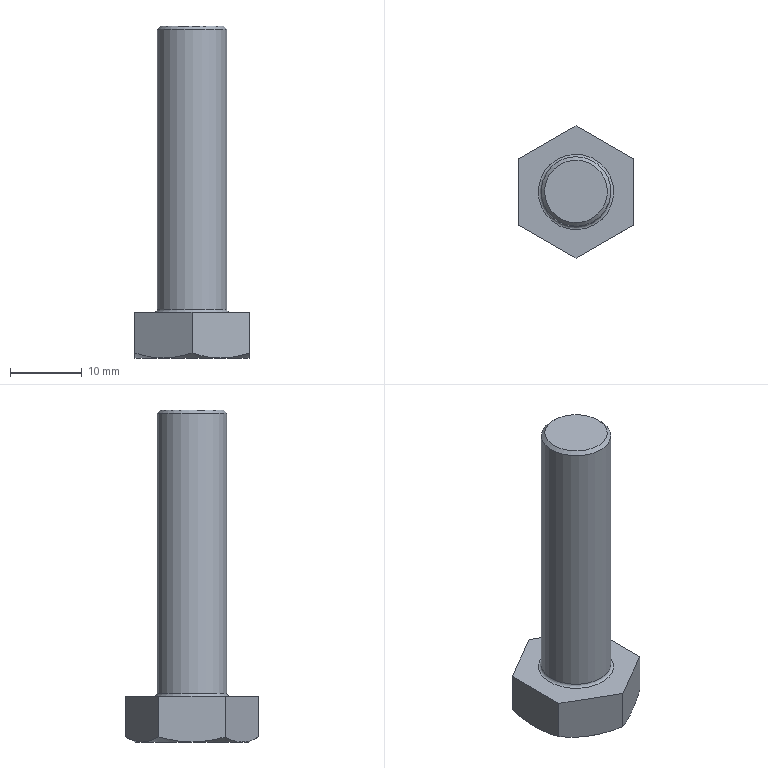Component | NX | GB-T5781-2000_M10X40 | 1 solid | 18 faces | volume 4387 mm3 | plane 9 | cone 7 | cylinder 1 | torus 1 | commonest cylinder face diameters 9.732 x1